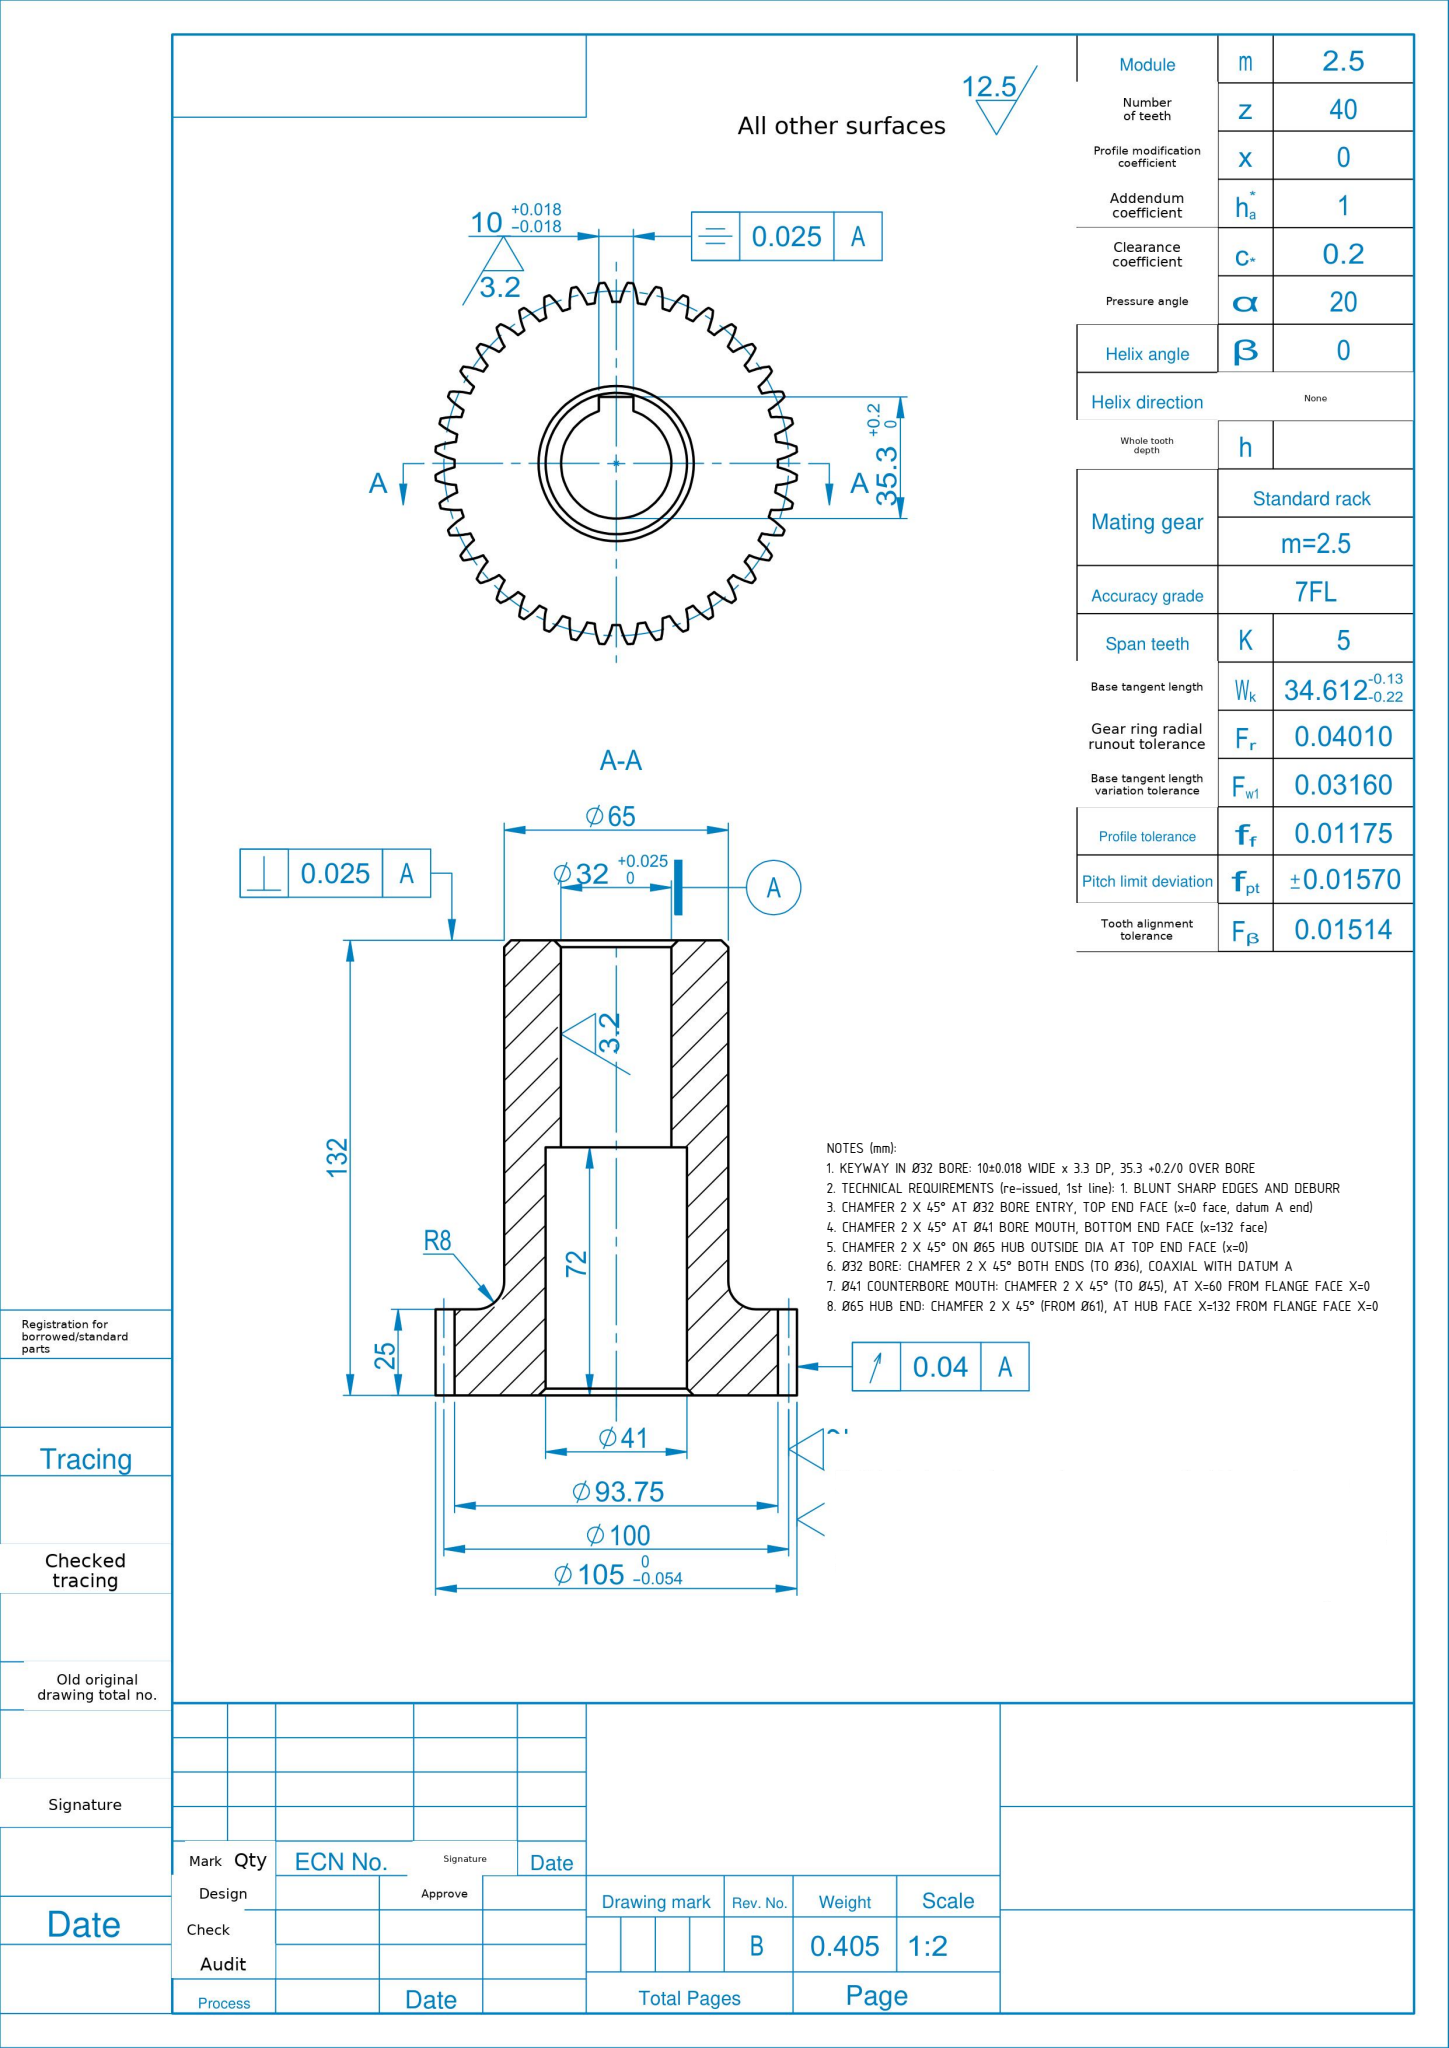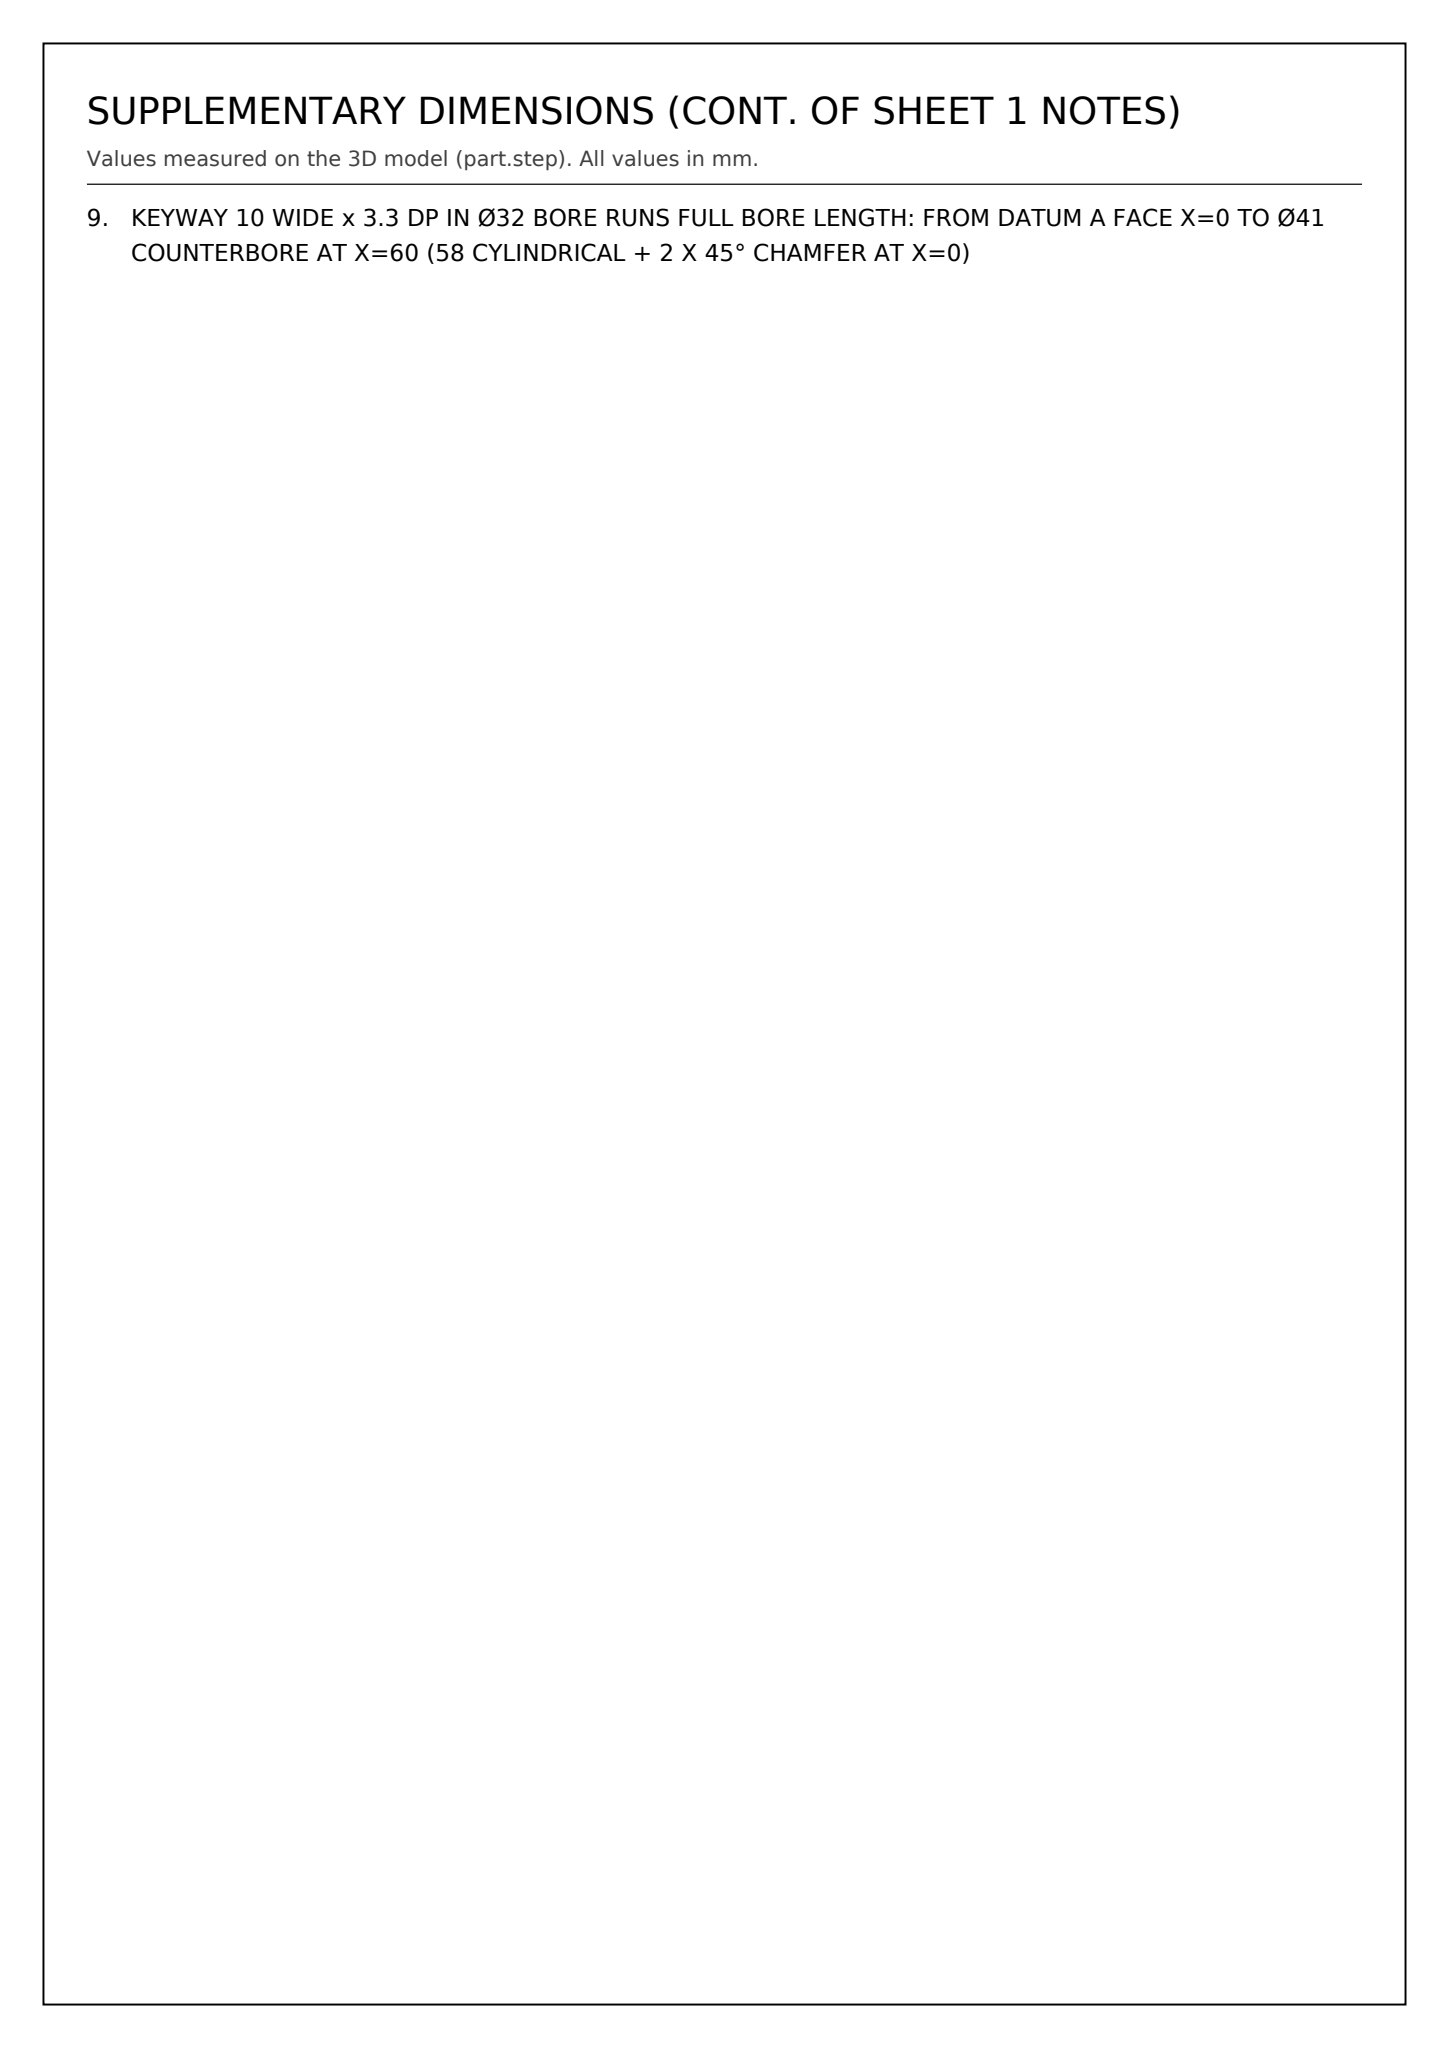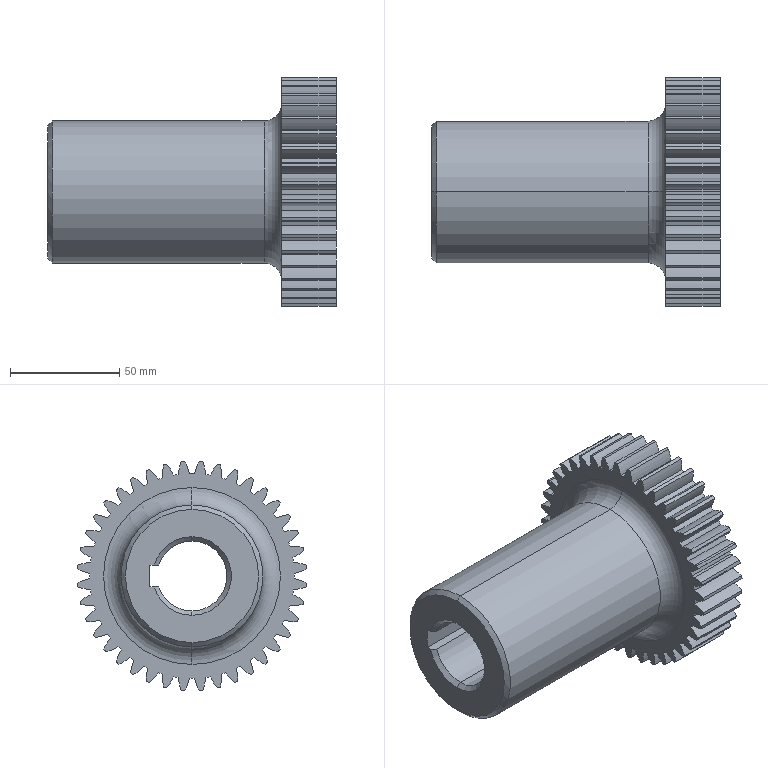Part | SolidWorks | mm | 1 solid | 188 faces | box 132 x 104.79 x 104.79 mm | volume 404920 mm3 | cylinder 172 | cone 7 | plane 7 | torus 2 | commonest cylinder face diameters 40 x84 93.748 x41 105 x40 32 x3 41 x2 65 x2
Drawing notes:
KEYWAY IN Ø32 BORE: 10±0.018 WIDE x 3.3 DP, 35.3 +0.2/0 OVER BORE | from the solid: Bore Ø32 axis at y=52.39,z=52.39; keyway flanks z=47.39 & z=57.39 (10 wide, centered); floor plane y=71.69 = 3.3 above bore top (y=68.39), 35.3 from opposite bore wall
TECHNICAL REQUIREMENTS (re-issued, 1st line): 1. BLUNT SHARP EDGES AND DEBURR | from the solid: text block continuation on sheet; no STEP geometry conflict
CHAMFER 2 X 45° AT Ø32 BORE ENTRY, TOP END FACE (x=0 face, datum A end) | from the solid: cones[included_angle,ref_dia] = [90.0, 36.0] on Ø32 bore (cylinder Ø32, axis x)
CHAMFER 2 X 45° AT Ø41 BORE MOUTH, BOTTOM END FACE (x=132 face) | from the solid: cones[included_angle,ref_dia] = [90.0, 41.0] at Ø41 bore end
CHAMFER 2 X 45° ON Ø65 HUB OUTSIDE DIA AT TOP END FACE (x=0) | from the solid: cones[included_angle,ref_dia] = [90.0, 61.0] on Ø65 hub, axis_planes x=0.0
Ø32 BORE: CHAMFER 2 X 45° BOTH ENDS (TO Ø36), COAXIAL WITH DATUM A | from the solid: cones[included_angle,ref_dia] = [90.0, 36.0] (3 instances) on Ø32 bore, axis x
Ø41 COUNTERBORE MOUTH: CHAMFER 2 X 45° (TO Ø45), AT X=60 FROM FLANGE FACE X=0 | from the solid: cones[included_angle,ref_dia] = [90.0, 41.0] (2 instances); axis_planes x=60.0 (Ø41/Ø32 step)
Ø65 HUB END: CHAMFER 2 X 45° (FROM Ø61), AT HUB FACE X=132 FROM FLANGE FACE X=0 | from the solid: cones[included_angle,ref_dia] = [90.0, 61.0] (2 instances); axis_planes x=0.0 and x=132.0 give 132 overall length
KEYWAY 10 WIDE x 3.3 DP IN Ø32 BORE RUNS FULL BORE LENGTH: FROM DATUM A FACE X=0 TO Ø41 COUNTERBORE AT X=60 (58 CYLINDRICAL + 2 X 45° CHAMFER AT X=0) | from the solid: cylinder Ø32 along x, length 58.0 (3 segments split by keyway); axis_planes x=0.0 and x=60.0; keyway flank planes z=47.39 and z=57.39 (10.0 apart); keyway floor plane y=71.69 vs bore axis y=52.39 (19.3 = 16 + 3.3); cone 90° ref_dia 36.0
build123d program:
from build123d import *

# Parameters (mm, degrees)
BASPROSKE_W        = 25
BASPROSKE_H        = 52.5
TOOTHCUT_DEPTH     = 79.342
TEETHCUTS_COUNT    = 40
TEETHCUTS_ANGLE    = 351
HUBNEAONESKE_R     = 32.5
HUBNEARONE_DEPTH   = 107
BORSKE_R           = 16
BORE_DEPTH         = 126
KEYSKE_W           = 10
KEYSKE_H           = 19.3
KEYWAY_DEPTH       = 126
SKETCH1_R          = 20.5
CUT_EXTRUDE1_DEPTH = 72
FILLET1_R          = 8
CHAMFER1_SIZE      = 2
CHAMFER2_SIZE      = 2


with BuildPart() as part:
    # BasProSke → Base-Revolve (revolve)
    with BuildSketch(Plane(origin=(0, 0, 0), x_dir=(1, 0, 0), z_dir=(0, 1, 0)), mode=Mode.PRIVATE) as base_revolve_sk:
        with Locations((12.5, 26.25)):
            Rectangle(BASPROSKE_W, BASPROSKE_H)
    revolve(base_revolve_sk.sketch.rotate(Axis((-10, 0, 0), (1, 0, 0)), 180), axis=Axis((-10, 0, 0), (1, 0, 0)))

    # TooCutSke → ToothCut (cut, through all)
    with BuildSketch(Plane(origin=(0, 0, 0), x_dir=(0, 0, -1), z_dir=(1, 0, 0))):
        with BuildLine():
            ThreePointArc((1.109, 46.861), (0, 46.874), (-1.109, 46.861))
            ThreePointArc((-1.109, 46.861), (-2.02, 49.724), (-3.35, 52.418))
            ThreePointArc((-3.35, 52.418), (0, 52.525), (3.35, 52.418))
            ThreePointArc((3.35, 52.418), (2.02, 49.724), (1.109, 46.861))
        make_face()
    toothcut = extrude(amount=TOOTHCUT_DEPTH, mode=Mode.SUBTRACT)

    # TeethCuts: ToothCut ×40 about axis
    teethcuts_axis = Axis((-10, 0, 0), (1, 0, 0))
    for i in range(1, TEETHCUTS_COUNT):
        add(toothcut.rotate(teethcuts_axis, i * TEETHCUTS_ANGLE / (TEETHCUTS_COUNT - 1)), mode=Mode.SUBTRACT)

    # HubNeaOneSke → HubNearOne (add)
    with BuildSketch(Plane.ZY):
        with Locations(Location((0, 0, 0), (0, 0, 180))):
            Circle(HUBNEAONESKE_R)
    extrude(amount=HUBNEARONE_DEPTH)

    # BorSke → Bore (cut, symmetric)
    with BuildSketch(Plane(origin=(0, 0, 0), x_dir=(0, 0, -1), z_dir=(1, 0, 0))):
        with Locations(Location((0, 0, 0), (0, 0, 180))):
            Circle(BORSKE_R)
    extrude(amount=BORE_DEPTH, both=True, mode=Mode.SUBTRACT)

    # KeySke → Keyway (cut, symmetric)
    with BuildSketch(Plane(origin=(0, 0, 0), x_dir=(0, 0, -1), z_dir=(1, 0, 0))):
        with Locations((0, 9.65)):
            Rectangle(KEYSKE_W, KEYSKE_H)
    extrude(amount=KEYWAY_DEPTH, both=True, mode=Mode.SUBTRACT)

    # Sketch1 → Cut-Extrude1 (cut)
    with BuildSketch(Plane(origin=(25, 0, 0), x_dir=(0, 0, -1), z_dir=(1, 0, 0))):
        Circle(SKETCH1_R)
    extrude(amount=-CUT_EXTRUDE1_DEPTH, mode=Mode.SUBTRACT)

    # Fillet1
    fillet1_edges = [part.edges().sort_by_distance(p)[0] for p in [
        (0, 0, 32.5),
    ]]
    fillet(fillet1_edges, radius=FILLET1_R)

    # Chamfer1
    chamfer1_edges = [part.edges().sort_by_distance(p)[0] for p in [
        (-107, 0, 32.5),
    ]]
    chamfer(chamfer1_edges, length=CHAMFER1_SIZE)

    # Chamfer2
    chamfer2_edges = [part.edges().sort_by_distance(p)[0] for p in [
        (-107, -16, 0),
        (25, 0, 20.5),
    ]]
    chamfer(chamfer2_edges, length=CHAMFER2_SIZE)


solid = part.part